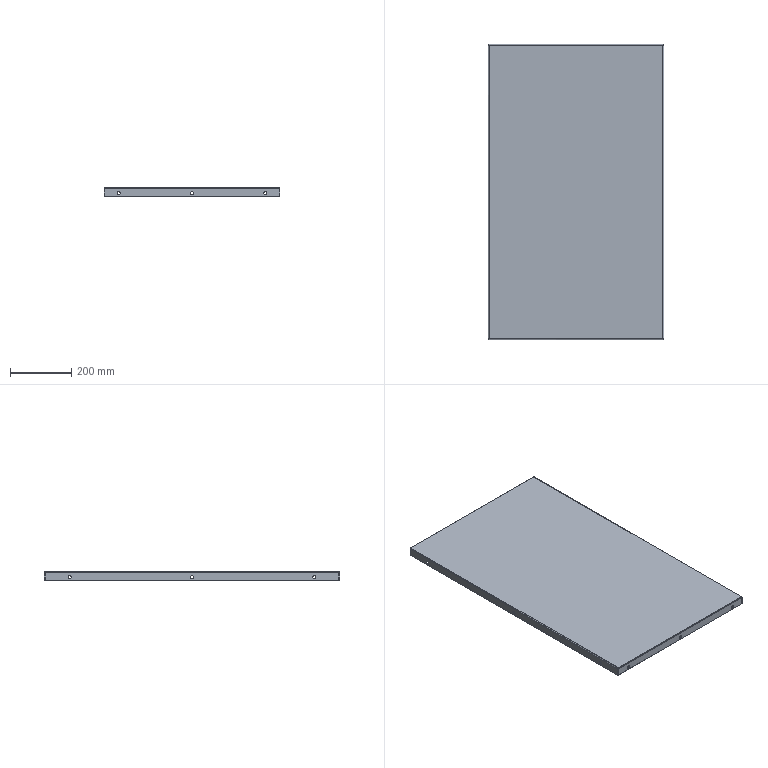Component | SolidWorks | 32FrontDoorUpperLeftPlate-2 | 1 solid | 62 faces | volume 1261814 mm3 | cylinder 32 | plane 22 | spline 8 | commonest cylinder face diameters 10 x24 2 x4 6 x4